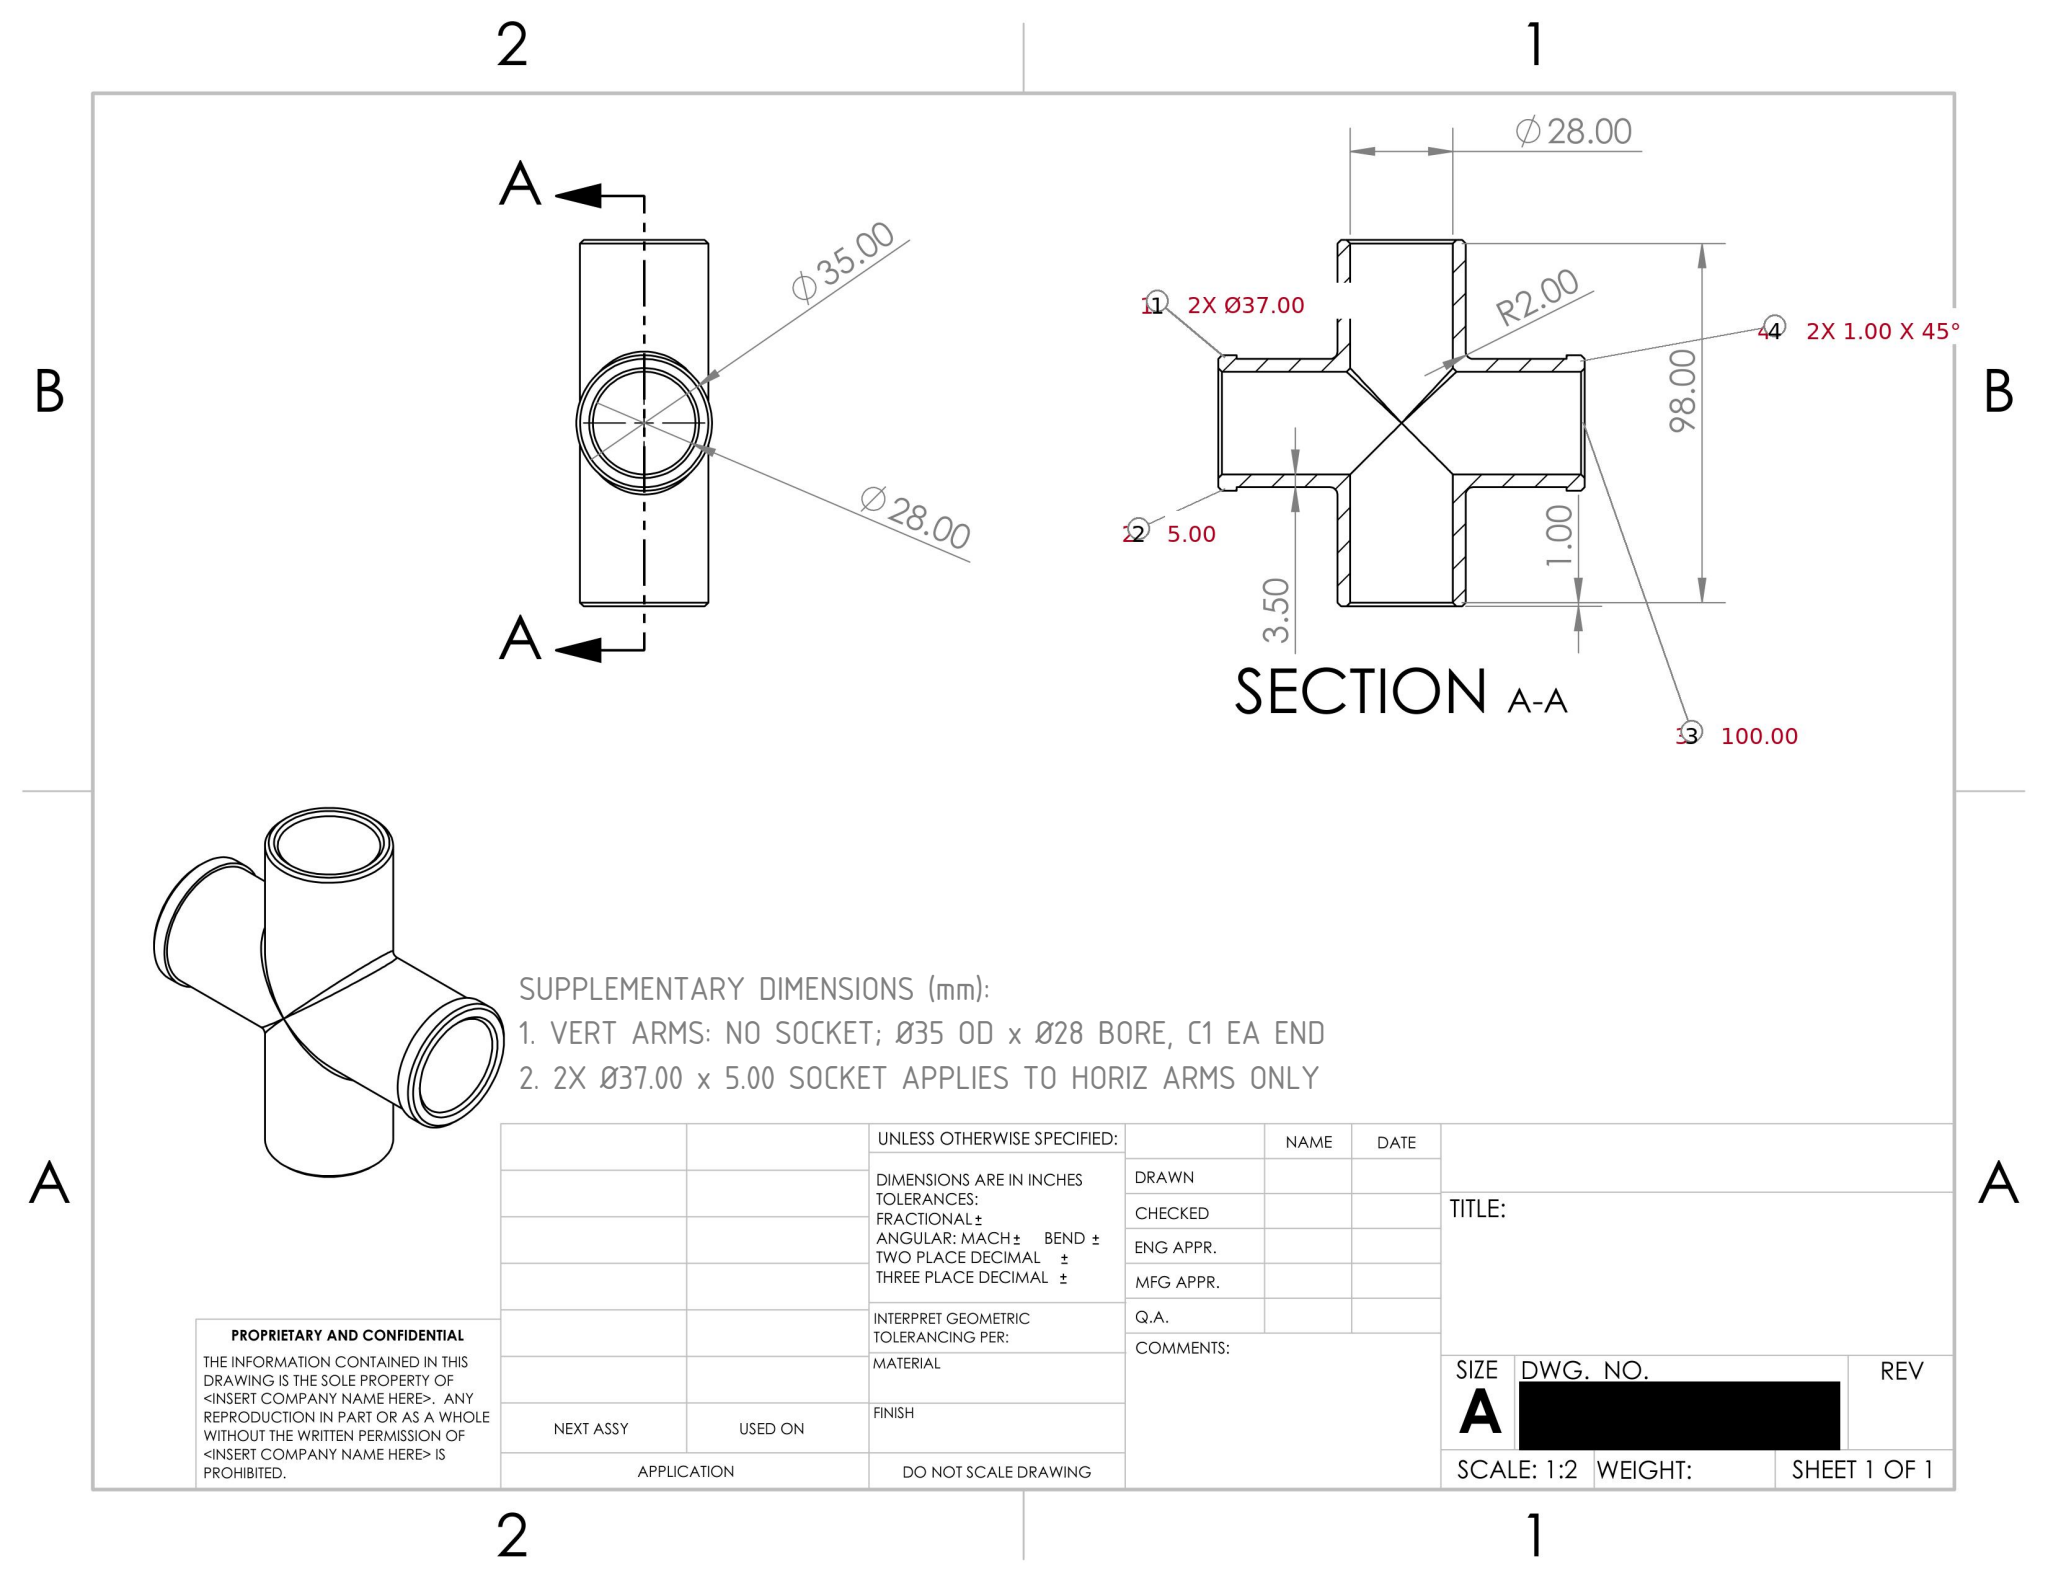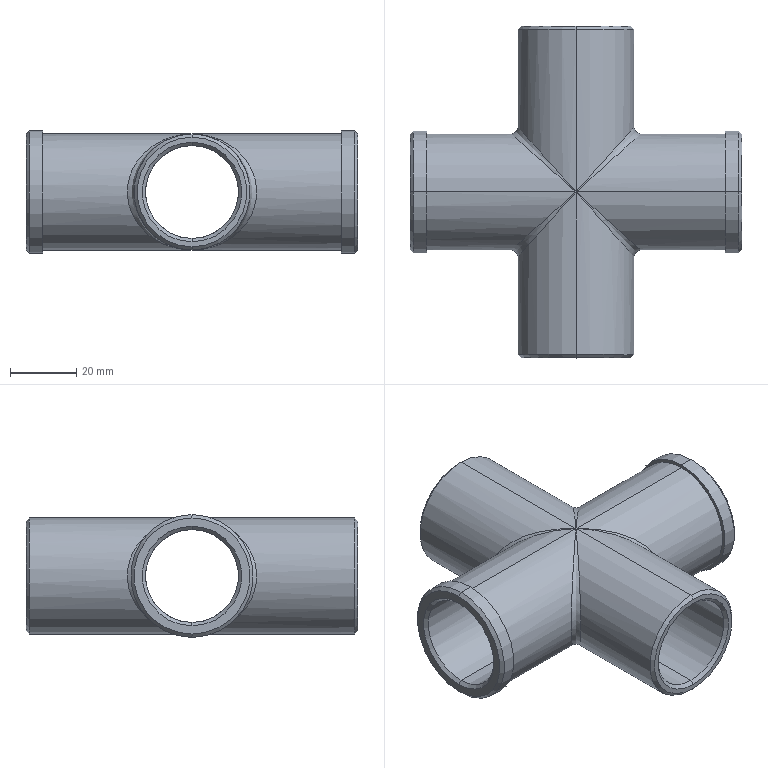Part | SolidWorks | mm | 1 solid | 48 faces | box 100 x 100 x 37 mm | volume 55994 mm3 | cylinder 20 | cone 16 | plane 6 | spline 6 | commonest cylinder face diameters 28 x8 35 x8 37 x4